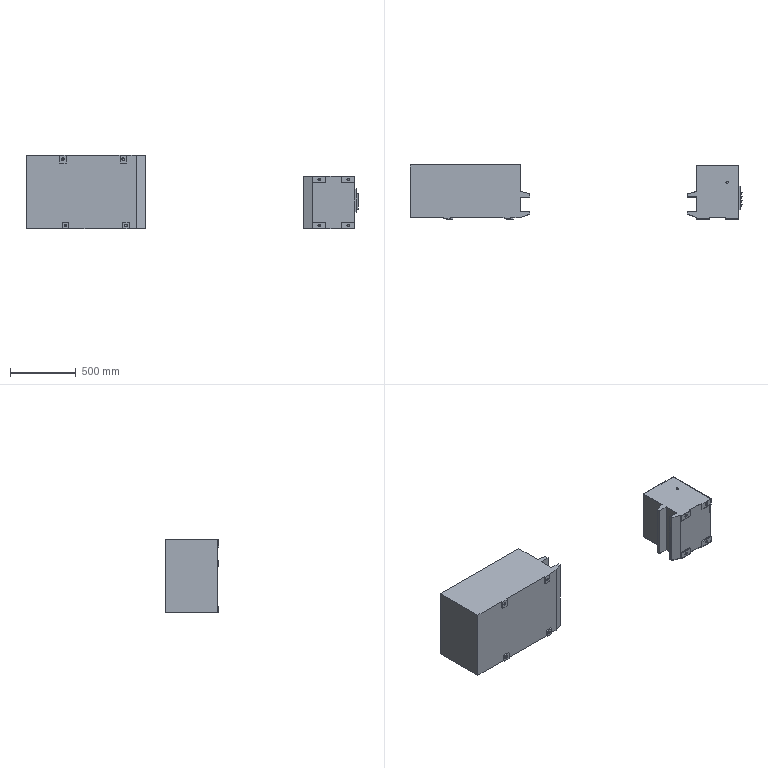Component | NX | LATHE_BASE | 2 solids | 190 faces | volume 192875555 mm3 | plane 142 | cone 24 | cylinder 24 | commonest cylinder face diameters 17.5 x8 82.165 x7 21.5 x4 78.165 x4 17 x1